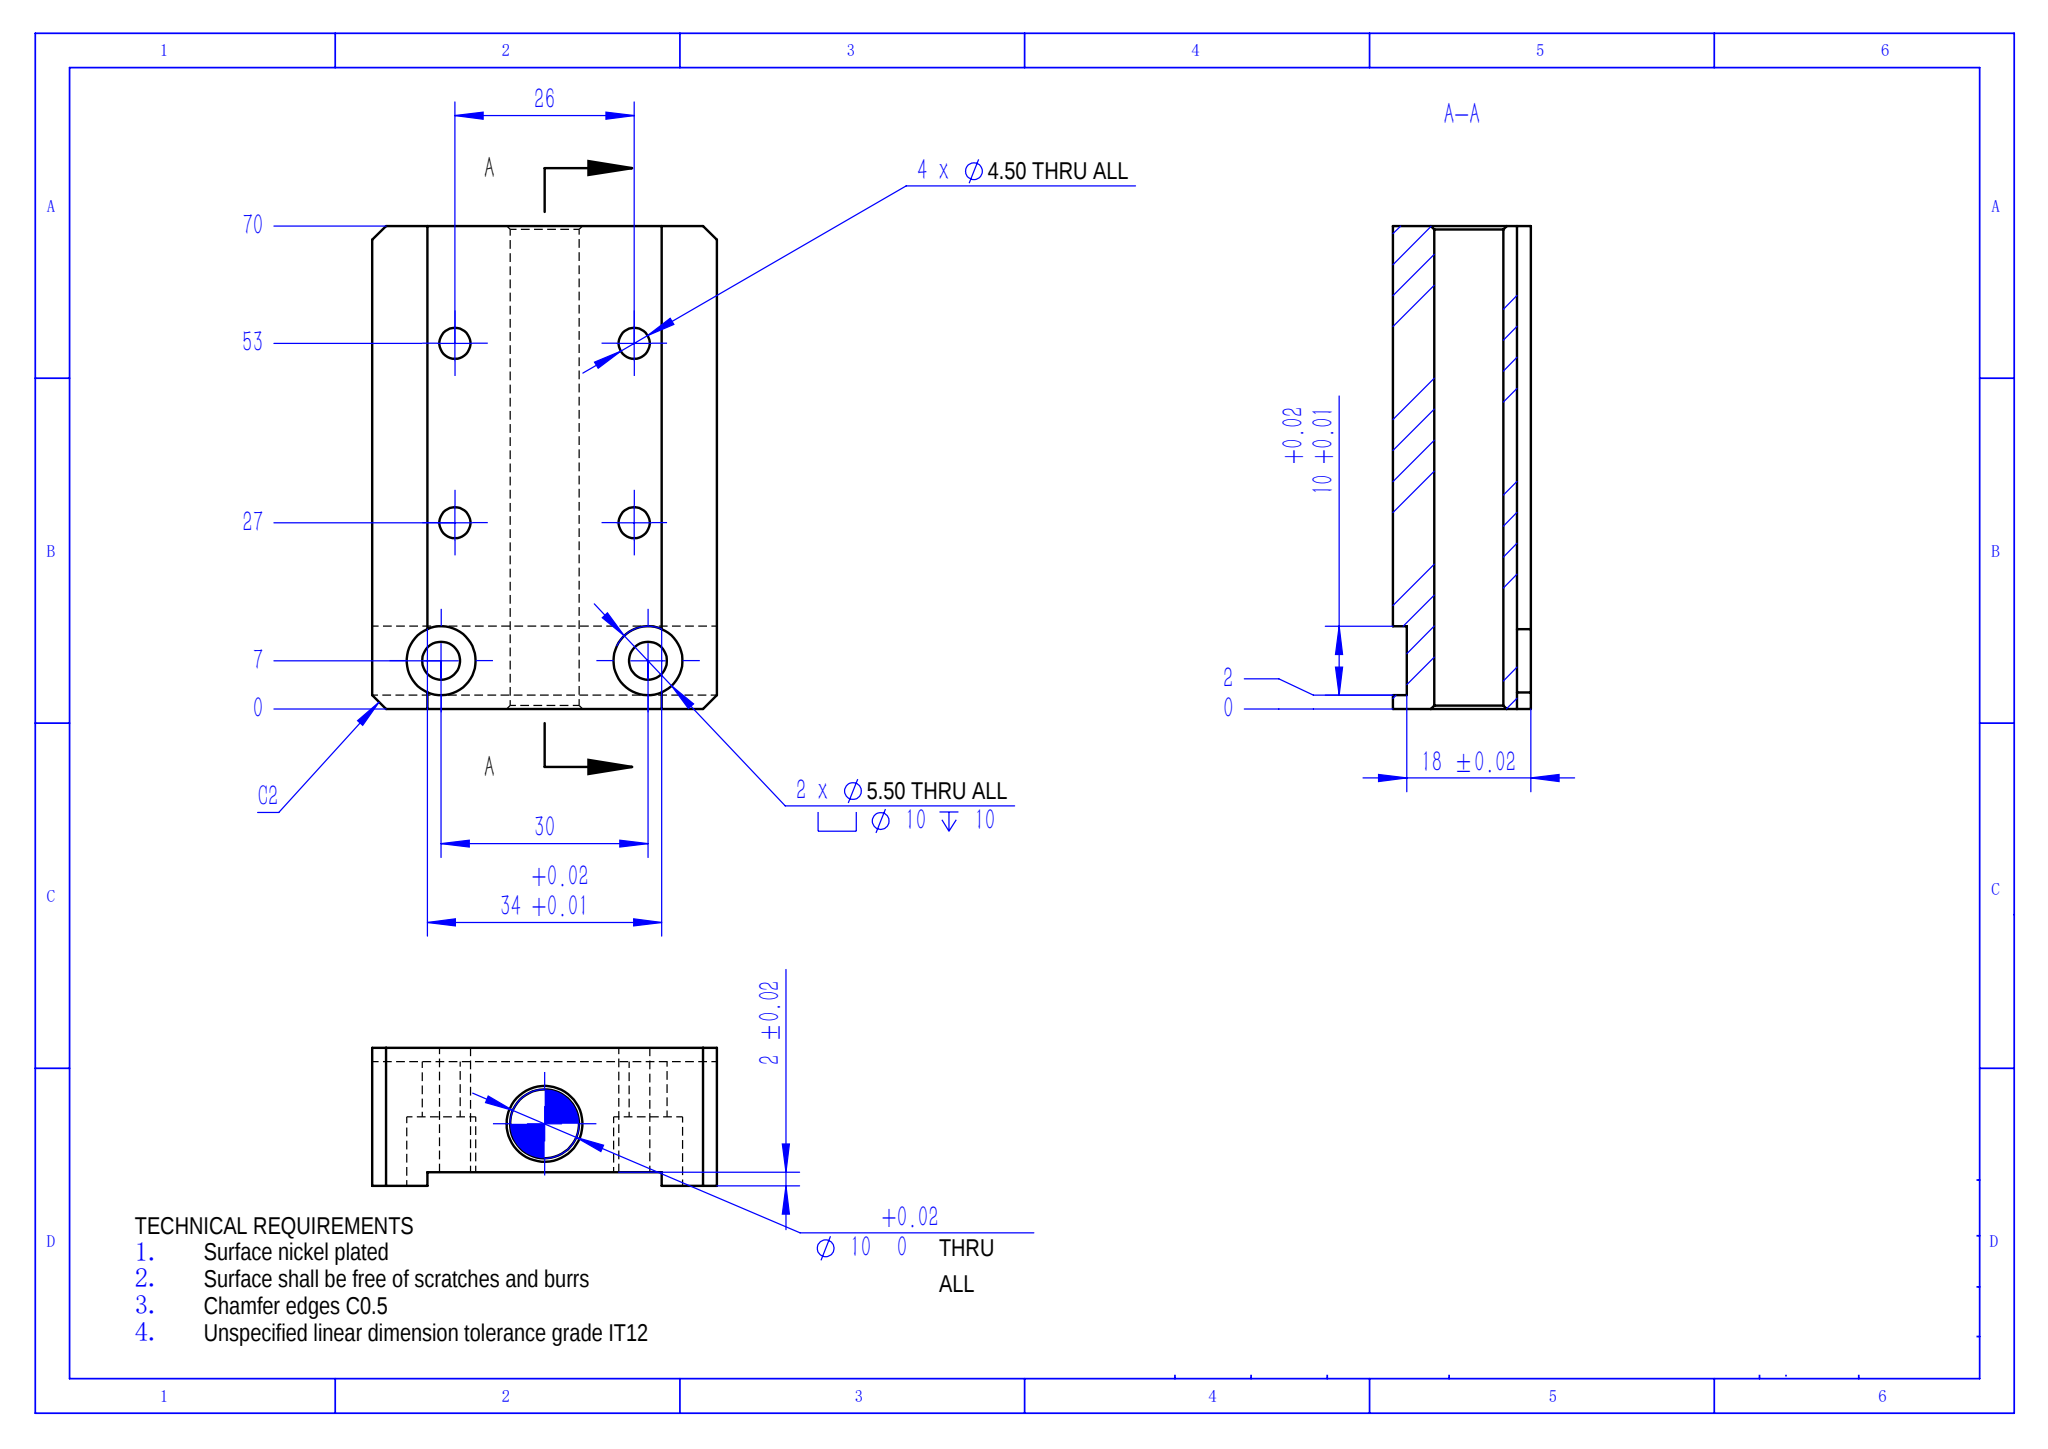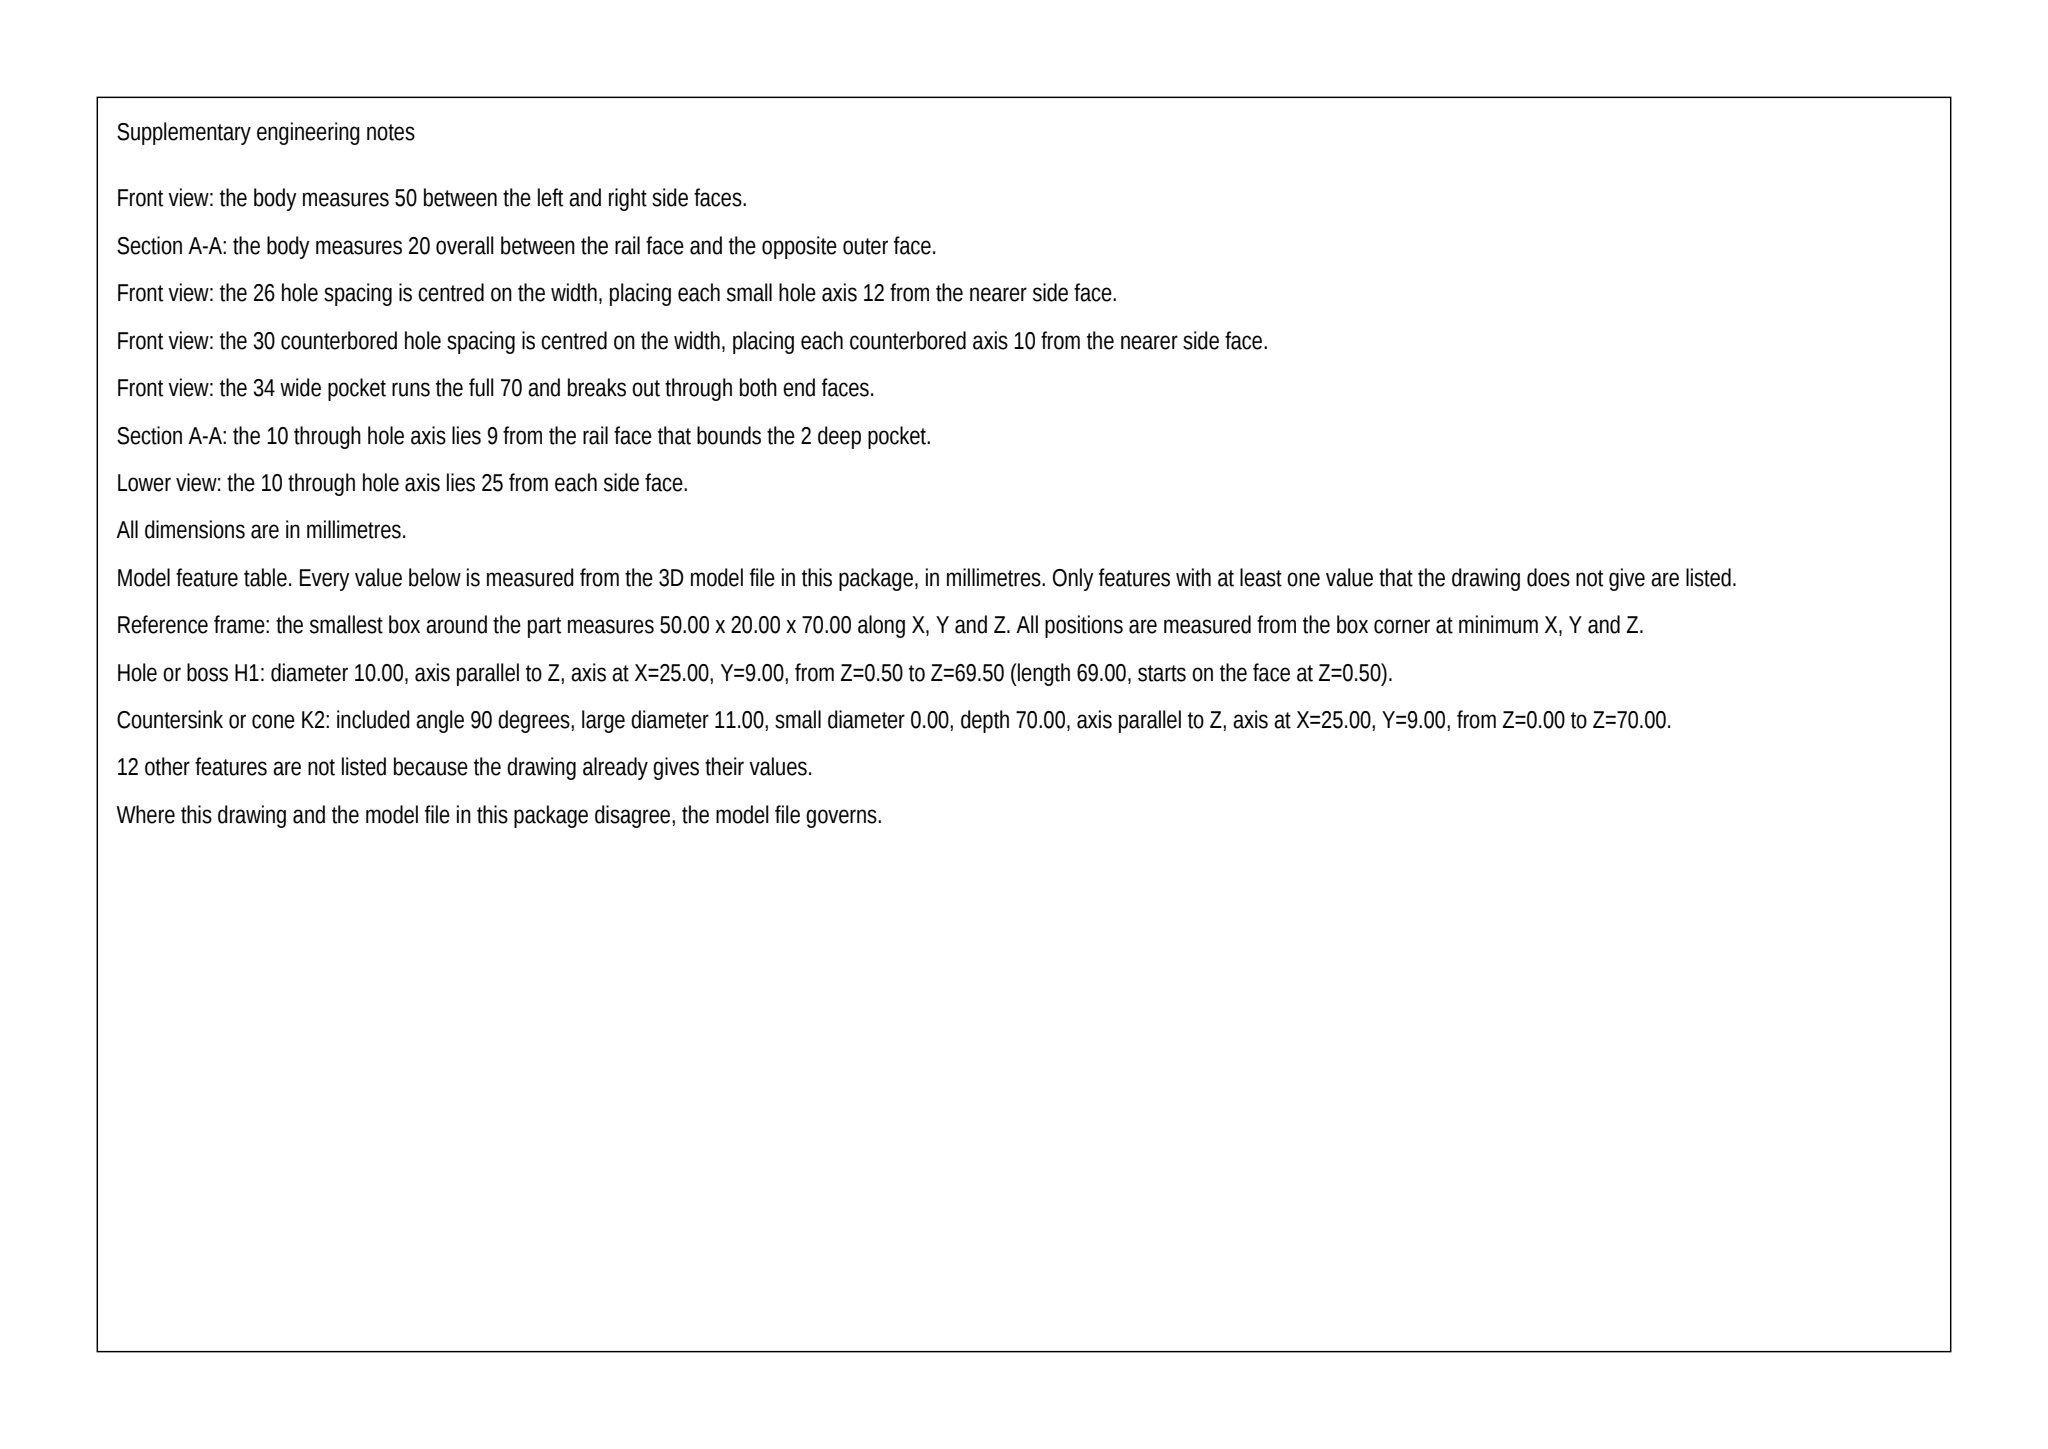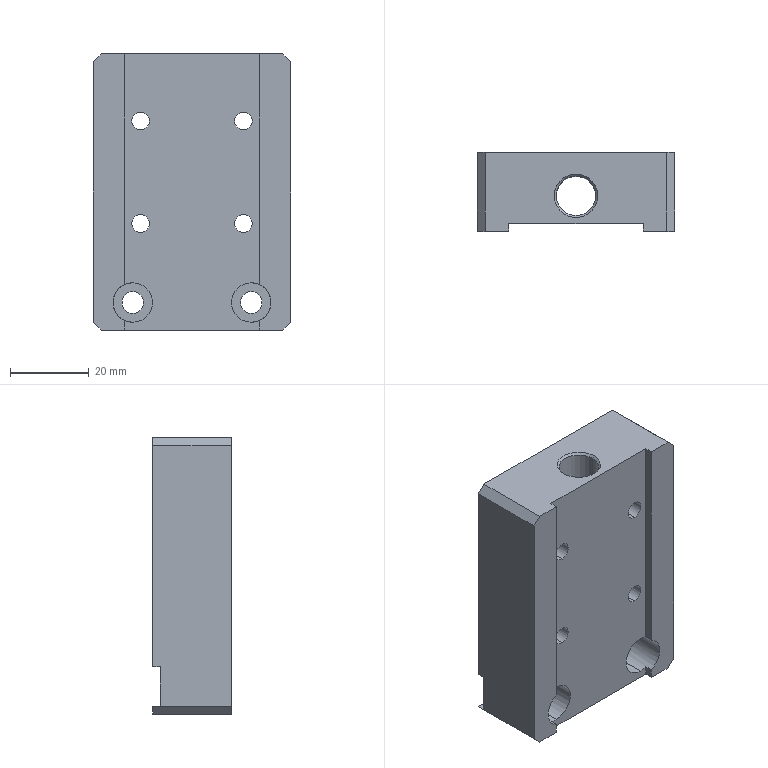Part | SolidWorks | mm | 1 solid | 44 faces | box 50 x 20 x 70 mm | volume 55713 mm3 | plane 22 | cylinder 18 | cone 4 | commonest cylinder face diameters 4.5 x8 10 x6 5.5 x4